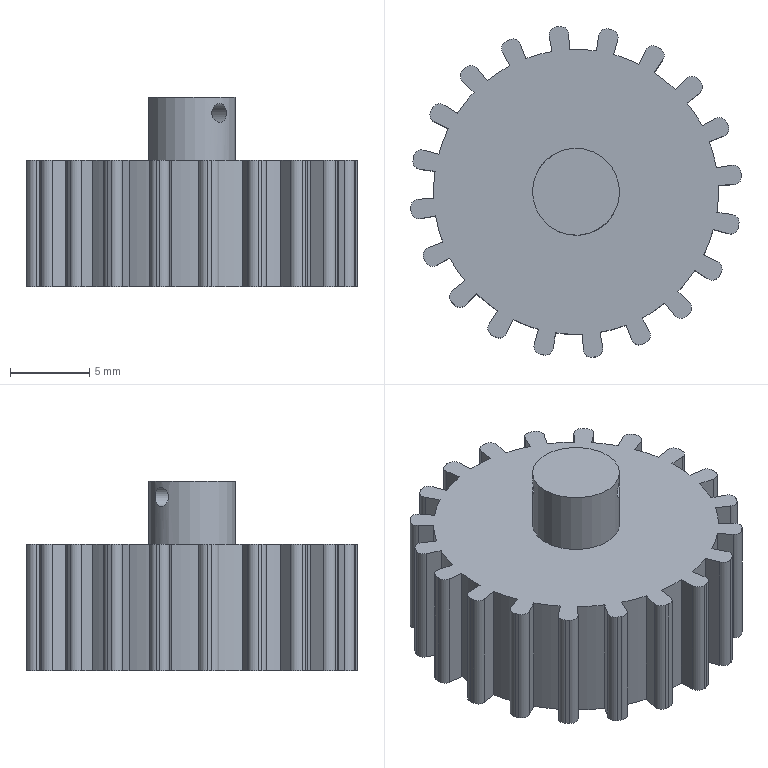Component | NX | GEAR_1 | 2 solids | 127 faces | volume 2272 mm3 | cylinder 83 | plane 44 | commonest cylinder face diameters 1 x40 21 x20 18 x20 5.5 x2 1.2 x1